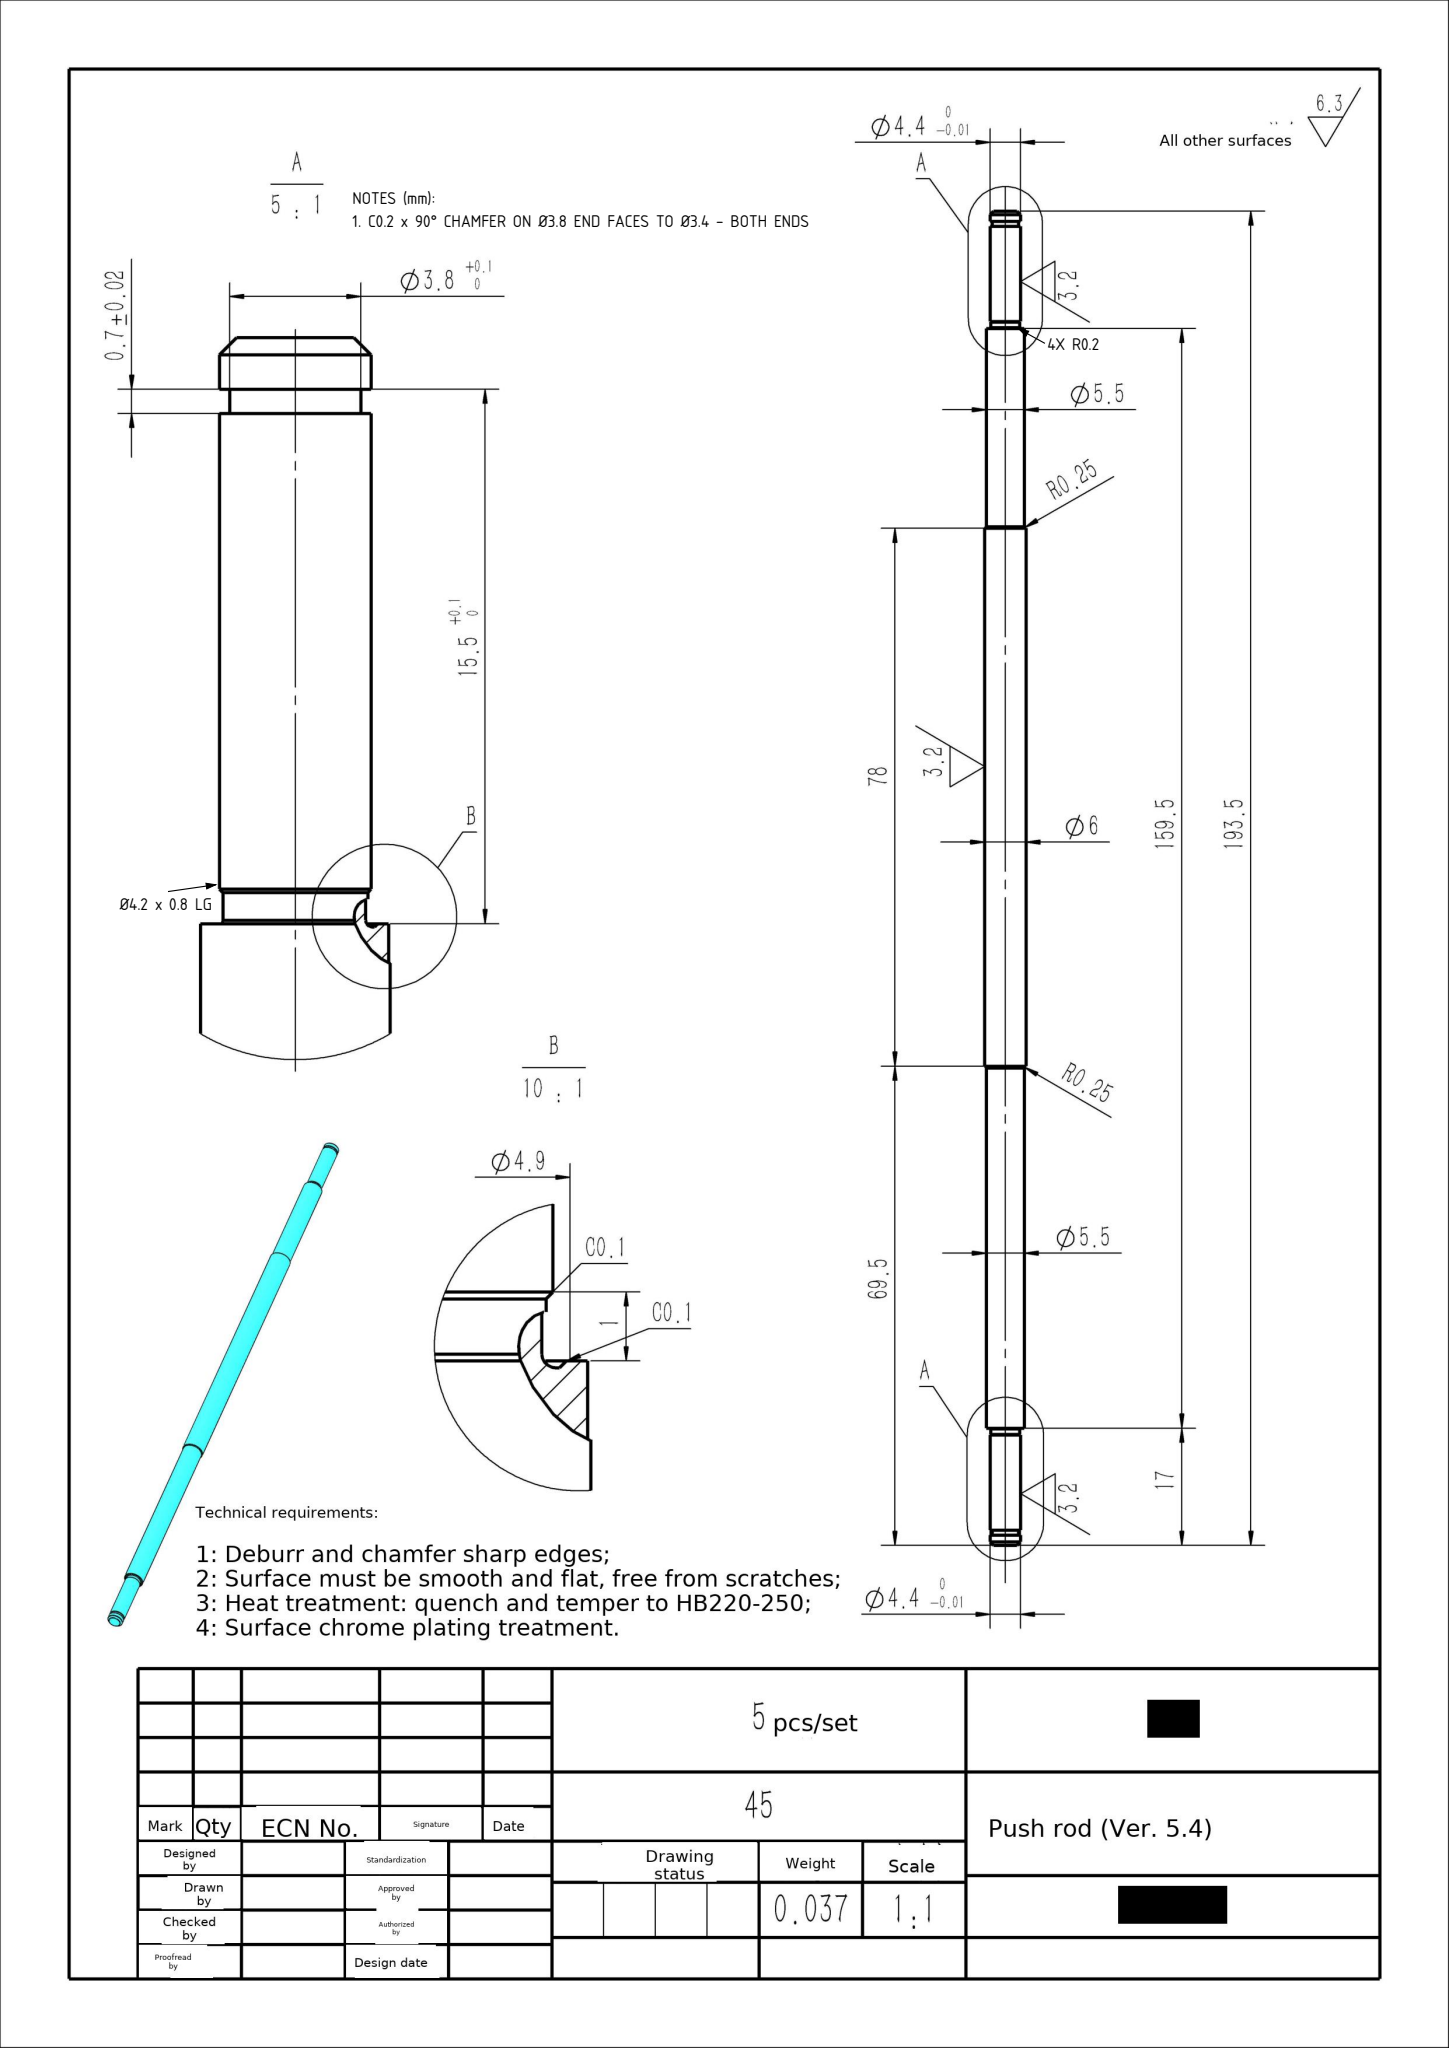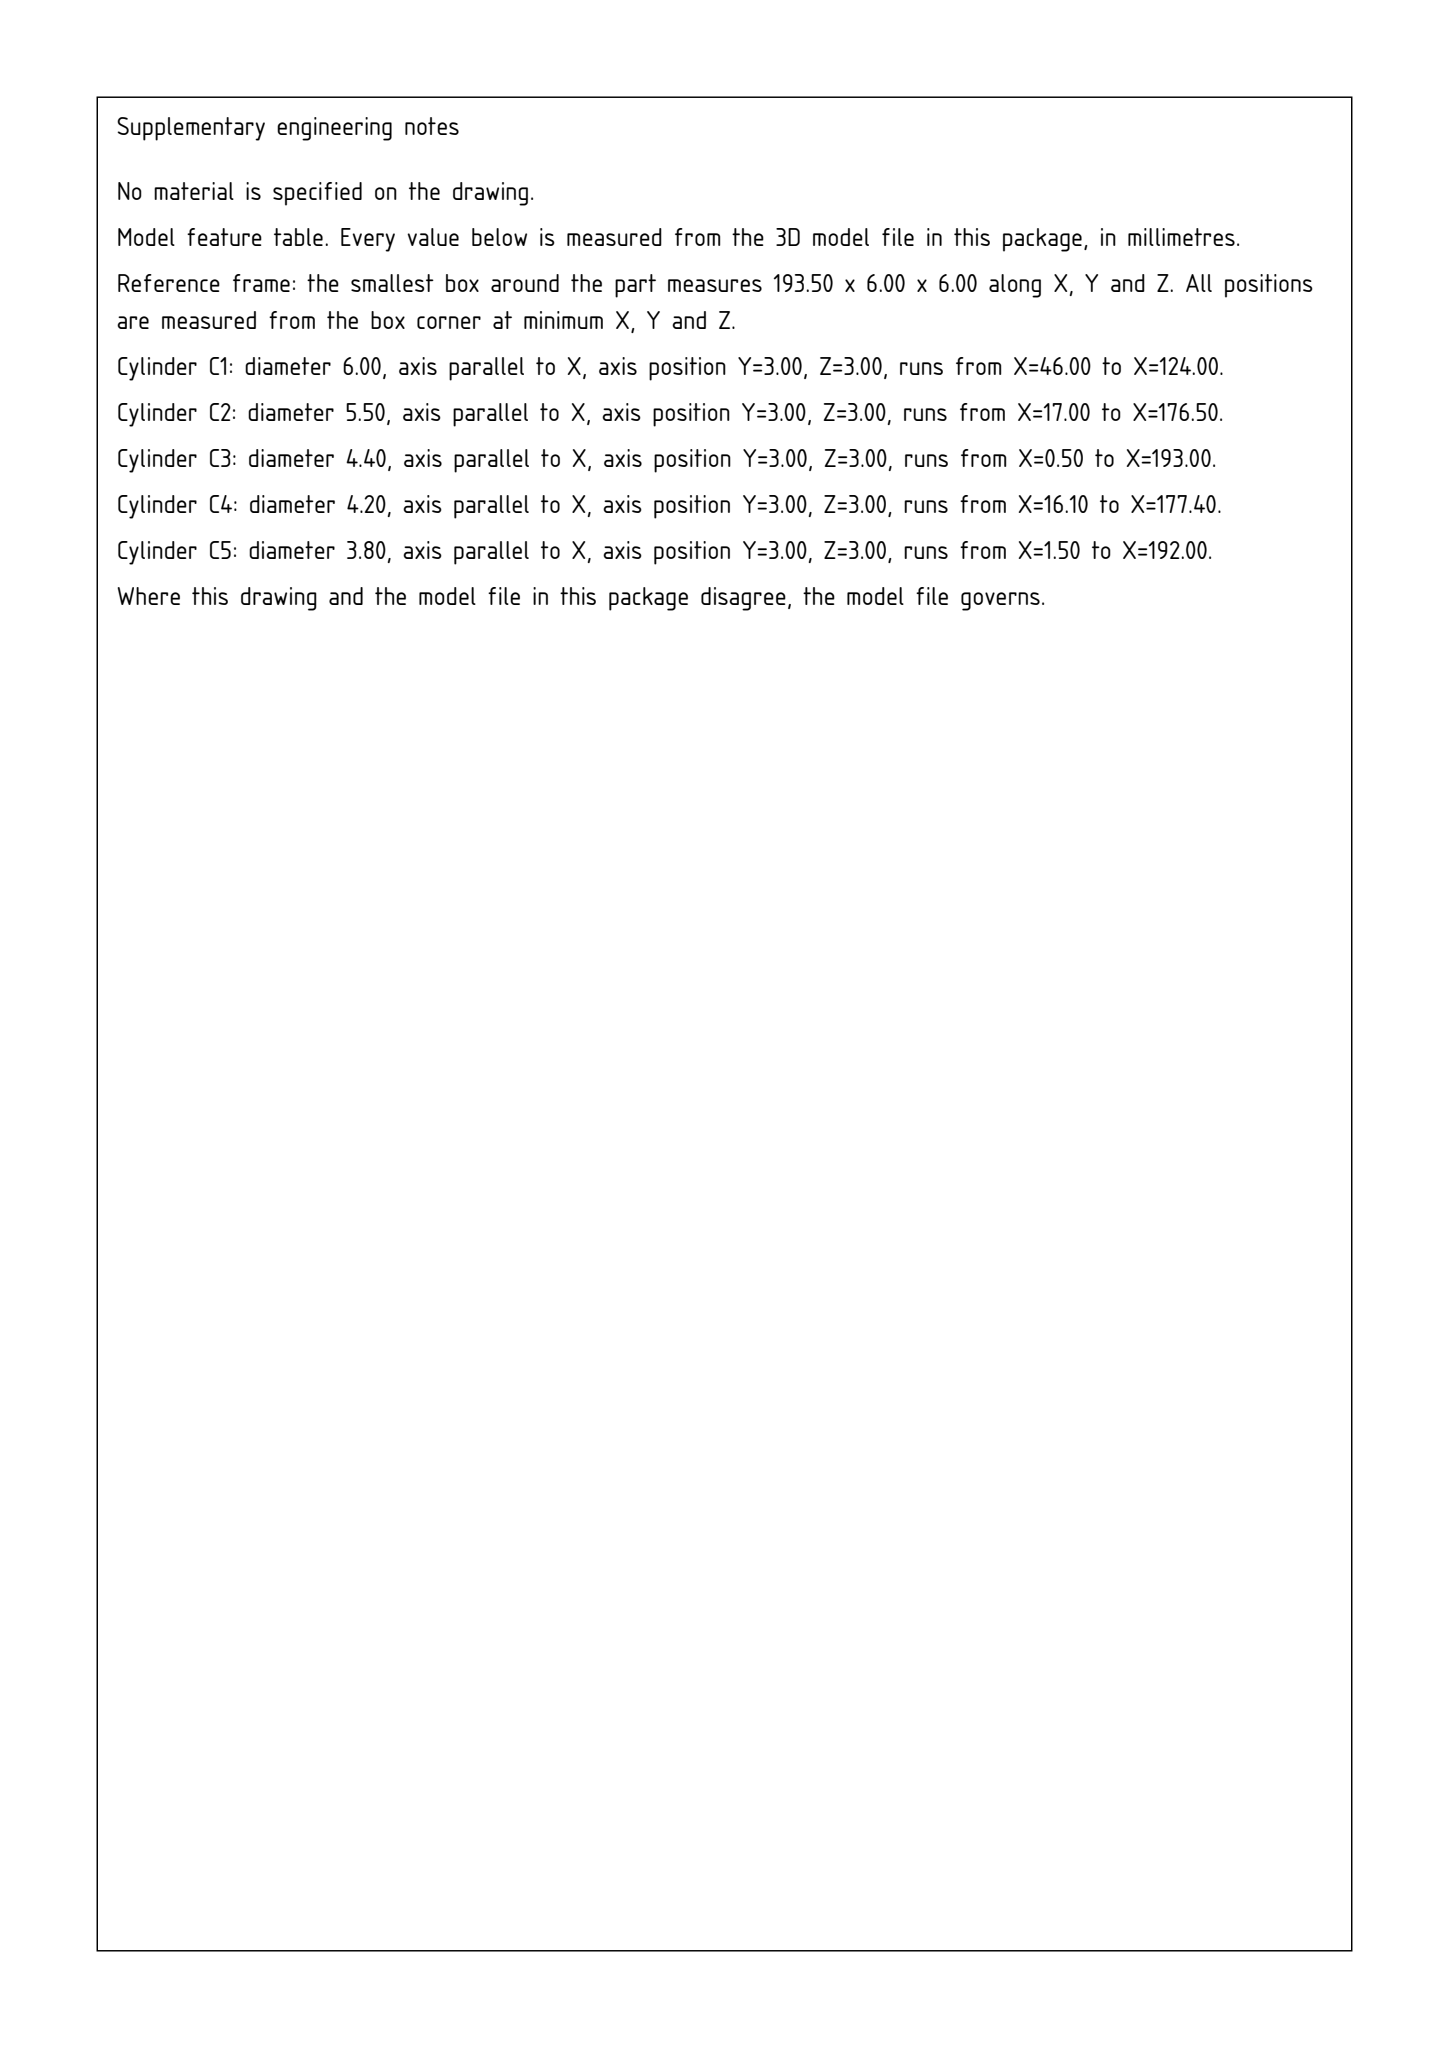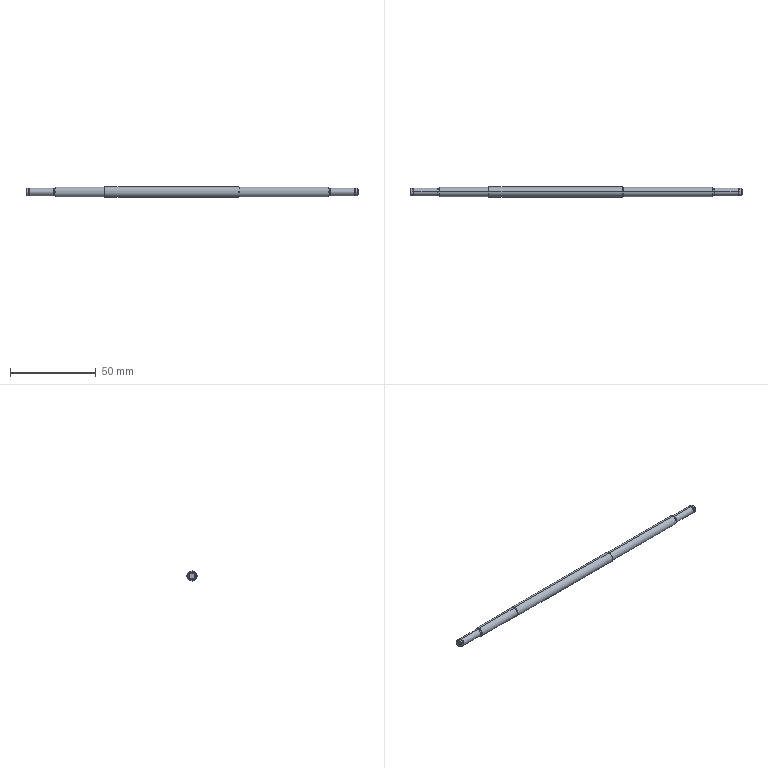Part | SolidWorks | mm | material 45 | 1 solid | 52 faces | box 193.5 x 6 x 6 mm | volume 4647 mm3 | cylinder 22 | cone 12 | plane 10 | torus 8 | commonest cylinder face diameters 4.4 x8 3.8 x4 4.2 x4 5.5 x4 6 x2
Drawing notes:
Ø4.2 STEP BETWEEN Ø3.8 TIP AND Ø4.4, 0.8 LG, 0.7 TO 1.5 FROM END FACE - BOTH ENDS | from the solid: cylinders Ø3.8x0.7, Ø4.2x0.8, Ø4.4x1.0 coaxial each end (4 off); x-planes 0.0, 1.5
C0.2 x 90° CHAMFER ON Ø3.8 END FACES TO Ø3.4 - BOTH ENDS | from the solid: cones 90° included angle, ref dia 3.4, 2 off at Ø3.8 ends
R0.2 AT Ø4.4/Ø5.5 SHOULDERS - 4 PL | from the solid: fillet_radii [0.2, 4] at Ø4.4/Ø5.5 steps